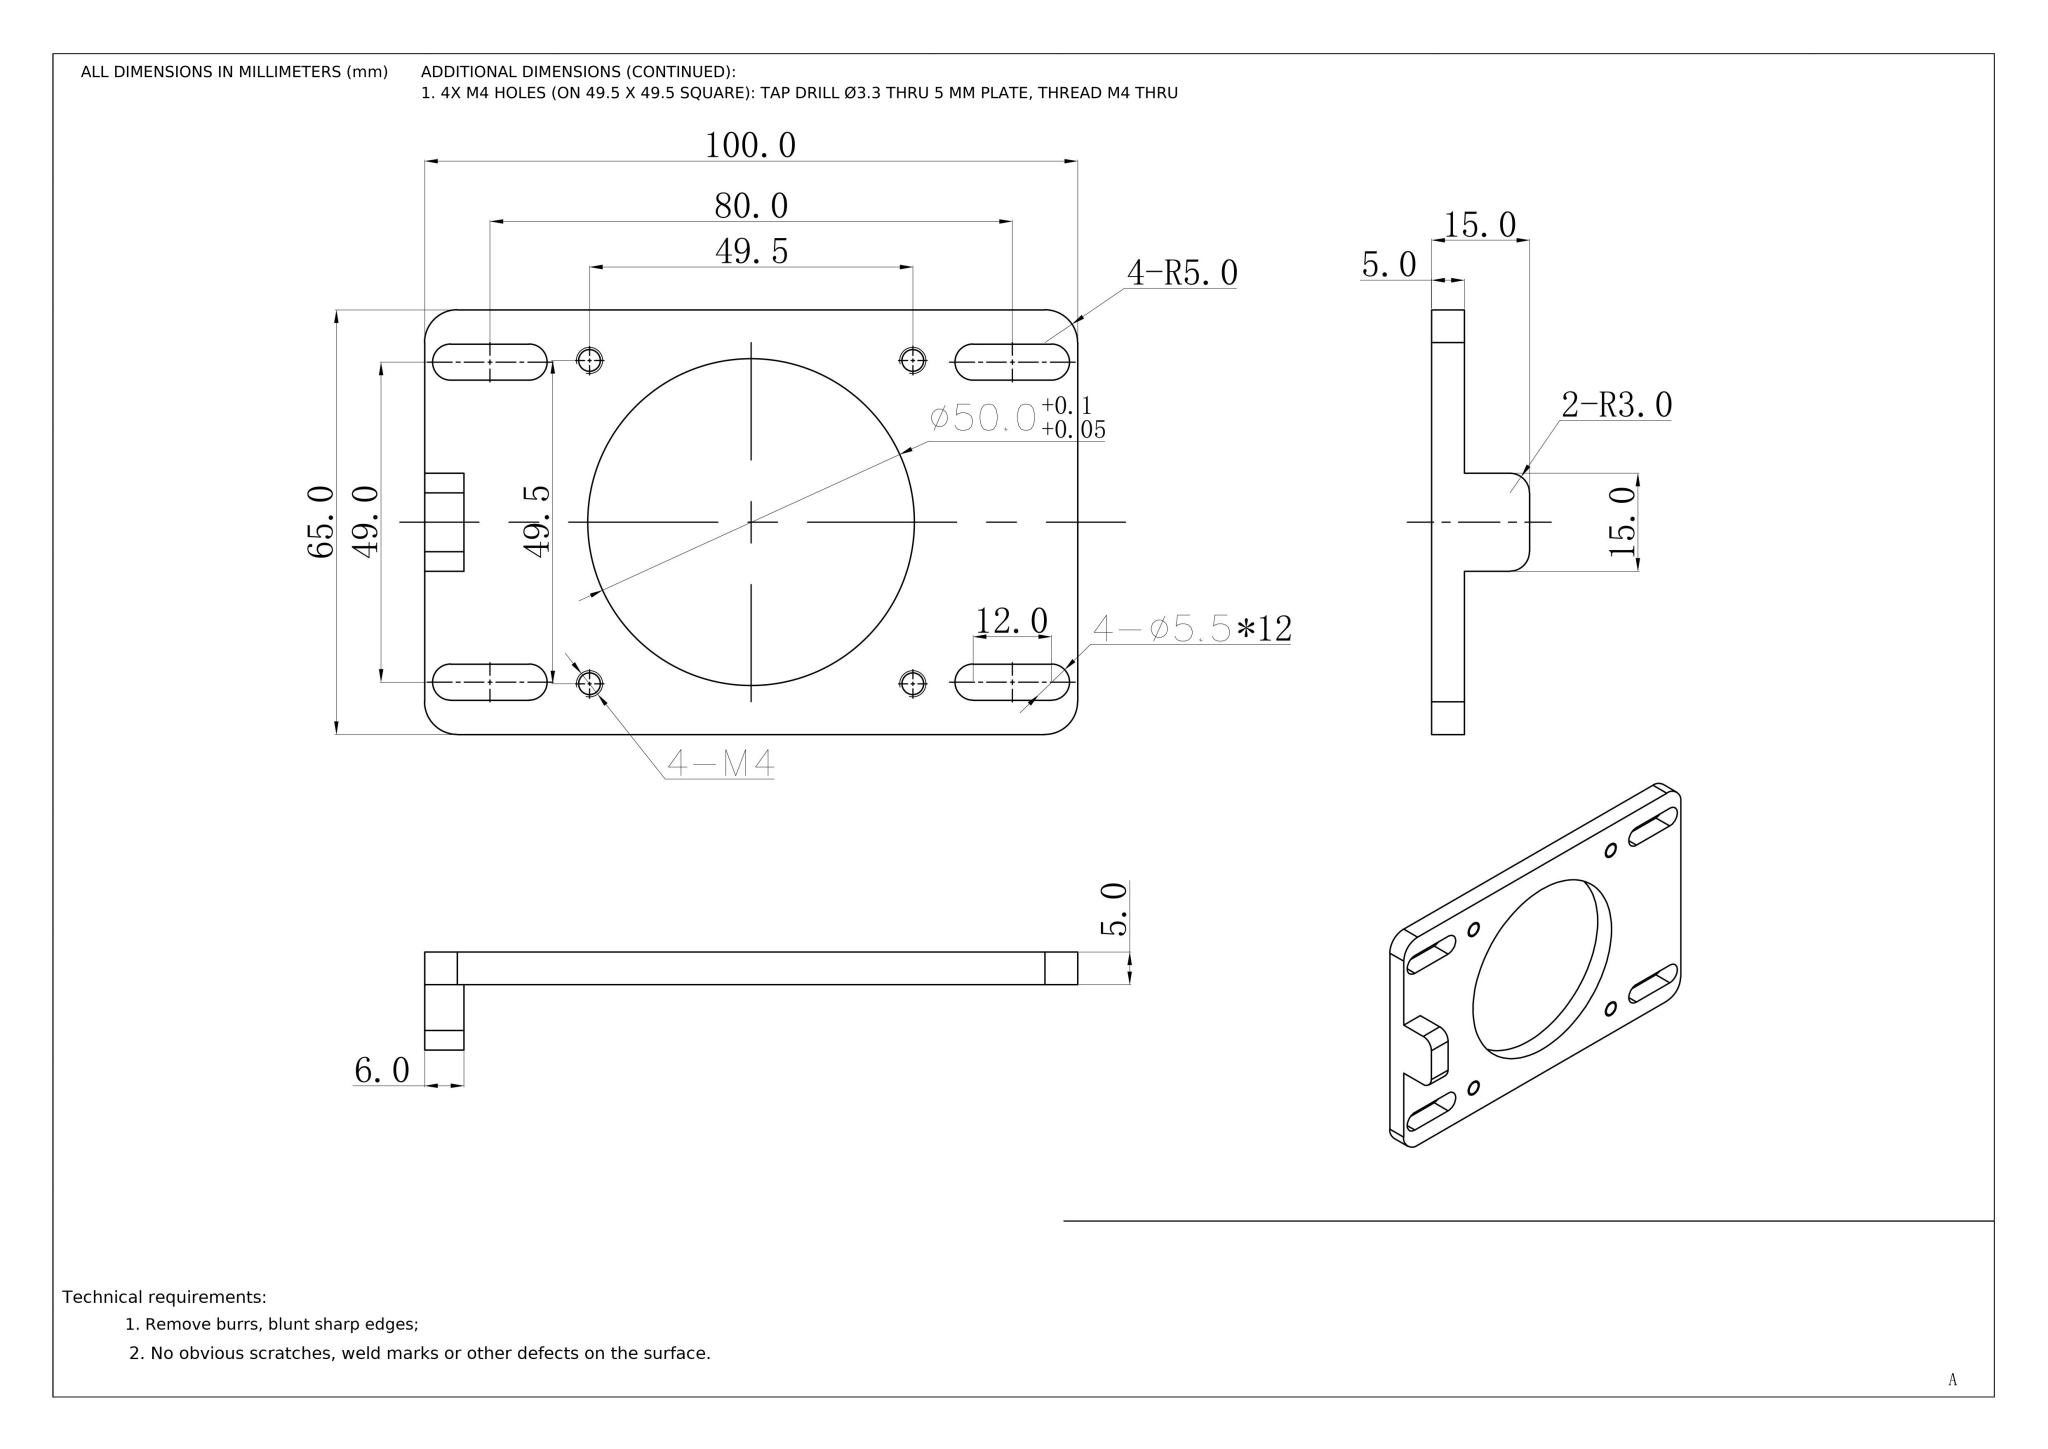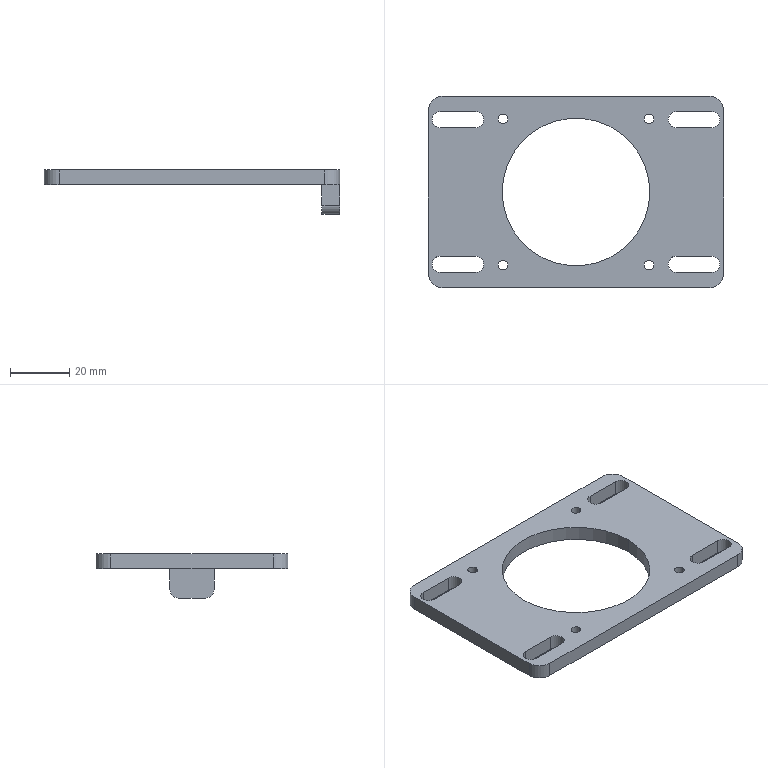Part | NX | mm | 1 solid | 46 faces | box 100 x 65 x 15 mm | volume 21486 mm3 | cylinder 28 | plane 18 | commonest cylinder face diameters 5.5 x12 3.3 x8 10 x4 50 x2 6 x2